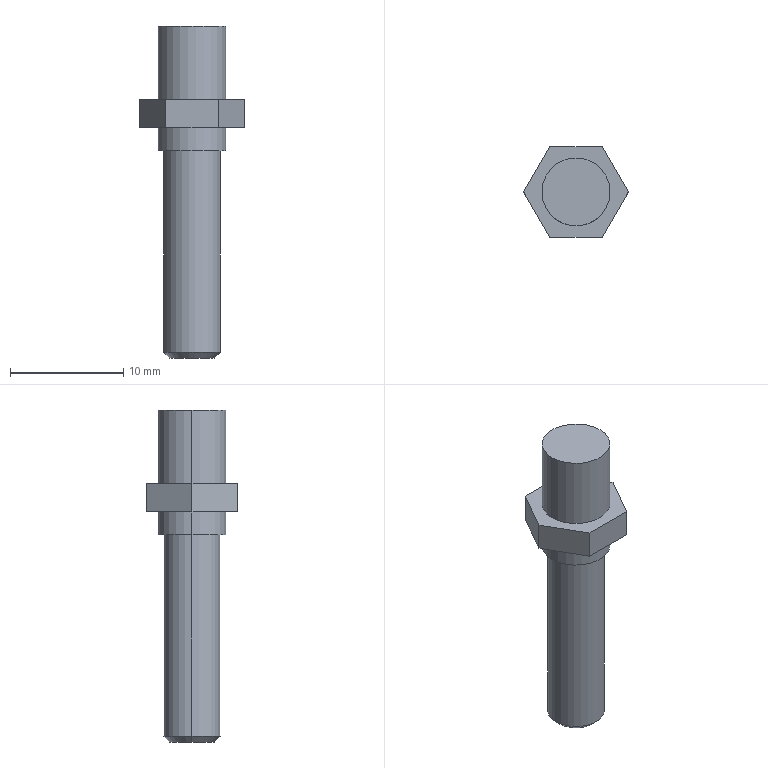Component | SolidWorks | CLS-MechanismAccessory5-1 | 1 solid | 19 faces | box 9.24 x 8 x 29.3 mm | volume 736 mm3 | plane 11 | cylinder 6 | cone 2 | commonest cylinder face diameters 6 x4 5 x2 | material 10 Cold Drawn Round Steel GB699-88
build123d program:
from build123d import *

# Parameters (mm, degrees)
BOSS_EXTRUDE1_DEPTH = 2.5
SKETCH2_R           = 3
BOSS_EXTRUDE2_DEPTH = 6.5
BOSS_EXTRUDE3_START = 2
SKETCH3_R           = 3
BOSS_EXTRUDE3_DEPTH = 2
SKETCH4_R           = 2.5
BOSS_EXTRUDE4_DEPTH = 18.3
CHAMFER1_SIZE       = 0.5


with BuildPart() as part:
    # Sketch1 → Boss-Extrude1 (new body)
    with BuildSketch(Plane.XY):
        Polygon((2.309, -4), (4.619, 0), (2.309, 4), (-2.309, 4), (-4.619, 0), (-2.309, -4), align=None)
    extrude(amount=BOSS_EXTRUDE1_DEPTH)

    # Sketch2 → Boss-Extrude2 (add)
    with BuildSketch(Plane.XY.offset(2.5)):
        with Locations(Location((0, 0, 0), (0, 0, 180))):
            Circle(SKETCH2_R)
    extrude(amount=BOSS_EXTRUDE2_DEPTH)

    # Sketch3 → Boss-Extrude3 (add)
    with BuildSketch(Plane(origin=(0, 0, 0), x_dir=(-1, 0, 0), z_dir=(0, 0, -1)).offset(BOSS_EXTRUDE3_START)):
        Circle(SKETCH3_R)
    extrude(amount=-BOSS_EXTRUDE3_DEPTH)

    # Sketch4 → Boss-Extrude4 (add)
    with BuildSketch(Plane(origin=(0, 0, -2), x_dir=(-1, 0, 0), z_dir=(0, 0, -1))):
        Circle(SKETCH4_R)
    extrude(amount=BOSS_EXTRUDE4_DEPTH)

    # Chamfer1
    chamfer1_edges = [part.edges().sort_by_distance(p)[0] for p in [
        (2.5, 0, -20.3),
    ]]
    chamfer(chamfer1_edges, length=CHAMFER1_SIZE)


solid = part.part

# Placed as in the assembly
solid = solid.moved(Location((63.64, 5.417, -1.001), (0, 0, 0)))
STEP:
#1=COLOUR_RGB('',0.7922,0.8196,0.9333);
#2=FILL_AREA_STYLE_COLOUR('',#1);
#3=FILL_AREA_STYLE('',(#2));
#4=SURFACE_STYLE_FILL_AREA(#3);
#5=SURFACE_SIDE_STYLE('',(#4));
#6=SURFACE_STYLE_USAGE(.BOTH.,#5);
#7=PRESENTATION_STYLE_ASSIGNMENT((#6));
#8=CARTESIAN_POINT('',(2.427,0.2133,-0.8386));
#9=VERTEX_POINT('',#8);
#10=CARTESIAN_POINT('',(2.584,0.2133,-0.8386));
#11=VERTEX_POINT('',#10);
#12=CARTESIAN_POINT('',(2.506,0.2133,-0.8386));
#13=DIRECTION('',(0.,0.,-1.));
#14=DIRECTION('',(-1.,0.,0.));
#15=AXIS2_PLACEMENT_3D('',#12,#13,#14);
#16=CIRCLE('',#15,0.07874);
#17=EDGE_CURVE('',#9,#11,#16,.T.);
#18=ORIENTED_EDGE('',*,*,#17,.F.);
#19=CARTESIAN_POINT('',(2.407,0.2133,-0.8189));
#20=VERTEX_POINT('',#19);
#21=CARTESIAN_POINT('',(2.427,0.2133,-0.8386));
#22=DIRECTION('',(-0.7071,0.,0.7071));
#23=VECTOR('',#22,39.37);
#24=LINE('',#21,#23);
#25=EDGE_CURVE('',#9,#20,#24,.T.);
#26=ORIENTED_EDGE('',*,*,#25,.T.);
#27=CARTESIAN_POINT('',(2.604,0.2133,-0.8189));
#28=VERTEX_POINT('',#27);
#29=CARTESIAN_POINT('',(2.506,0.2133,-0.8189));
#30=DIRECTION('',(0.,0.,1.));
#31=DIRECTION('',(-1.,0.,0.));
#32=AXIS2_PLACEMENT_3D('',#29,#30,#31);
#33=CIRCLE('',#32,0.09843);
#34=EDGE_CURVE('',#28,#20,#33,.T.);
#35=ORIENTED_EDGE('',*,*,#34,.F.);
#36=CARTESIAN_POINT('',(2.584,0.2133,-0.8386));
#37=DIRECTION('',(0.7071,0.,0.7071));
#38=VECTOR('',#37,39.37);
#39=LINE('',#36,#38);
#40=EDGE_CURVE('',#11,#28,#39,.T.);
#41=ORIENTED_EDGE('',*,*,#40,.F.);
#42=EDGE_LOOP('',(#18,#26,#35,#41));
#43=FACE_OUTER_BOUND('',#42,.T.);
#44=CARTESIAN_POINT('',(2.506,0.2133,-0.8386));
#45=DIRECTION('',(0.,0.,1.));
#46=DIRECTION('',(1.,0.,0.));
#47=AXIS2_PLACEMENT_3D('',#44,#45,#46);
#48=CONICAL_SURFACE('',#47,0.07874,0.7854);
#49=ADVANCED_FACE('',(#43),#48,.T.);
#50=ORIENTED_EDGE('',*,*,#34,.T.);
#51=CARTESIAN_POINT('',(2.407,0.2133,-0.1181));
#52=VERTEX_POINT('',#51);
#53=CARTESIAN_POINT('',(2.407,0.2133,-0.8386));
#54=DIRECTION('',(0.,0.,1.));
#55=VECTOR('',#54,39.37);
#56=LINE('',#53,#55);
#57=EDGE_CURVE('',#20,#52,#56,.T.);
#58=ORIENTED_EDGE('',*,*,#57,.T.);
#59=CARTESIAN_POINT('',(2.604,0.2133,-0.1181));
#60=VERTEX_POINT('',#59);
#61=CARTESIAN_POINT('',(2.506,0.2133,-0.1181));
#62=DIRECTION('',(0.,0.,-1.));
#63=DIRECTION('',(-1.,0.,0.));
#64=AXIS2_PLACEMENT_3D('',#61,#62,#63);
#65=CIRCLE('',#64,0.09843);
#66=EDGE_CURVE('',#52,#60,#65,.T.);
#67=ORIENTED_EDGE('',*,*,#66,.T.);
#68=CARTESIAN_POINT('',(2.604,0.2133,-0.8386));
#69=DIRECTION('',(0.,0.,1.));
#70=VECTOR('',#69,39.37);
#71=LINE('',#68,#70);
#72=EDGE_CURVE('',#28,#60,#71,.T.);
#73=ORIENTED_EDGE('',*,*,#72,.F.);
#74=EDGE_LOOP('',(#50,#58,#67,#73));
#75=FACE_OUTER_BOUND('',#74,.T.);
#76=CARTESIAN_POINT('',(2.506,0.2133,-0.8386));
#77=DIRECTION('',(0.,0.,1.));
#78=DIRECTION('',(1.,0.,0.));
#79=AXIS2_PLACEMENT_3D('',#76,#77,#78);
#80=CYLINDRICAL_SURFACE('',#79,0.09843);
#81=ADVANCED_FACE('',(#75),#80,.T.);
#82=CARTESIAN_POINT('',(2.387,0.2133,-0.1181));
#83=VERTEX_POINT('',#82);
#84=CARTESIAN_POINT('',(2.624,0.2133,-0.1181));
#85=VERTEX_POINT('',#84);
#86=CARTESIAN_POINT('',(2.506,0.2133,-0.1181));
#87=DIRECTION('',(0.,0.,-1.));
#88=DIRECTION('',(-1.,0.,0.));
#89=AXIS2_PLACEMENT_3D('',#86,#87,#88);
#90=CIRCLE('',#89,0.1181);
#91=EDGE_CURVE('',#83,#85,#90,.T.);
#92=ORIENTED_EDGE('',*,*,#91,.F.);
#93=CARTESIAN_POINT('',(2.387,0.2133,-0.03939));
#94=VERTEX_POINT('',#93);
#95=CARTESIAN_POINT('',(2.387,0.2133,-0.1181));
#96=DIRECTION('',(0.,0.,1.));
#97=VECTOR('',#96,39.37);
#98=LINE('',#95,#97);
#99=EDGE_CURVE('',#83,#94,#98,.T.);
#100=ORIENTED_EDGE('',*,*,#99,.T.);
#101=CARTESIAN_POINT('',(2.624,0.2133,-0.03939));
#102=VERTEX_POINT('',#101);
#103=CARTESIAN_POINT('',(2.506,0.2133,-0.03939));
#104=DIRECTION('',(0.,0.,-1.));
#105=DIRECTION('',(1.,0.,0.));
#106=AXIS2_PLACEMENT_3D('',#103,#104,#105);
#107=CIRCLE('',#106,0.1181);
#108=EDGE_CURVE('',#94,#102,#107,.T.);
#109=ORIENTED_EDGE('',*,*,#108,.T.);
#110=CARTESIAN_POINT('',(2.624,0.2133,-0.1181));
#111=DIRECTION('',(0.,0.,1.));
#112=VECTOR('',#111,39.37);
#113=LINE('',#110,#112);
#114=EDGE_CURVE('',#85,#102,#113,.T.);
#115=ORIENTED_EDGE('',*,*,#114,.F.);
#116=EDGE_LOOP('',(#92,#100,#109,#115));
#117=FACE_OUTER_BOUND('',#116,.T.);
#118=CARTESIAN_POINT('',(2.506,0.2133,-0.1181));
#119=DIRECTION('',(0.,0.,1.));
#120=DIRECTION('',(1.,0.,0.));
#121=AXIS2_PLACEMENT_3D('',#118,#119,#120);
#122=CYLINDRICAL_SURFACE('',#121,0.1181);
#123=ADVANCED_FACE('',(#117),#122,.T.);
#124=CARTESIAN_POINT('',(2.624,0.2133,0.3149));
#125=VERTEX_POINT('',#124);
#126=CARTESIAN_POINT('',(2.387,0.2133,0.3149));
#127=VERTEX_POINT('',#126);
#128=CARTESIAN_POINT('',(2.506,0.2133,0.3149));
#129=DIRECTION('',(0.,0.,1.));
#130=DIRECTION('',(1.,0.,0.));
#131=AXIS2_PLACEMENT_3D('',#128,#129,#130);
#132=CIRCLE('',#131,0.1181);
#133=EDGE_CURVE('',#125,#127,#132,.T.);
#134=ORIENTED_EDGE('',*,*,#133,.F.);
#135=CARTESIAN_POINT('',(2.624,0.2133,0.05903));
#136=VERTEX_POINT('',#135);
#137=CARTESIAN_POINT('',(2.624,0.2133,0.3149));
#138=DIRECTION('',(0.,0.,-1.));
#139=VECTOR('',#138,39.37);
#140=LINE('',#137,#139);
#141=EDGE_CURVE('',#125,#136,#140,.T.);
#142=ORIENTED_EDGE('',*,*,#141,.T.);
#143=CARTESIAN_POINT('',(2.387,0.2133,0.05903));
#144=VERTEX_POINT('',#143);
#145=CARTESIAN_POINT('',(2.506,0.2133,0.05903));
#146=DIRECTION('',(0.,0.,1.));
#147=DIRECTION('',(1.,0.,0.));
#148=AXIS2_PLACEMENT_3D('',#145,#146,#147);
#149=CIRCLE('',#148,0.1181);
#150=EDGE_CURVE('',#136,#144,#149,.T.);
#151=ORIENTED_EDGE('',*,*,#150,.T.);
#152=CARTESIAN_POINT('',(2.387,0.2133,0.3149));
#153=DIRECTION('',(0.,0.,-1.));
#154=VECTOR('',#153,39.37);
#155=LINE('',#152,#154);
#156=EDGE_CURVE('',#127,#144,#155,.T.);
#157=ORIENTED_EDGE('',*,*,#156,.F.);
#158=EDGE_LOOP('',(#134,#142,#151,#157));
#159=FACE_OUTER_BOUND('',#158,.T.);
#160=CARTESIAN_POINT('',(2.506,0.2133,0.3149));
#161=DIRECTION('',(0.,0.,-1.));
#162=DIRECTION('',(-1.,0.,0.));
#163=AXIS2_PLACEMENT_3D('',#160,#161,#162);
#164=CYLINDRICAL_SURFACE('',#163,0.1181);
#165=ADVANCED_FACE('',(#159),#164,.T.);
#166=CARTESIAN_POINT('',(2.506,0.2133,-0.1181));
#167=DIRECTION('',(0.,0.,-1.));
#168=DIRECTION('',(-1.,0.,0.));
#169=AXIS2_PLACEMENT_3D('',#166,#167,#168);
#170=CIRCLE('',#169,0.1181);
#171=EDGE_CURVE('',#85,#83,#170,.T.);
#172=ORIENTED_EDGE('',*,*,#171,.T.);
#173=ORIENTED_EDGE('',*,*,#91,.T.);
#174=EDGE_LOOP('',(#172,#173));
#175=FACE_OUTER_BOUND('',#174,.T.);
#176=CARTESIAN_POINT('',(2.506,0.2133,-0.1181));
#177=DIRECTION('',(0.,0.,-1.));
#178=DIRECTION('',(-1.,0.,0.));
#179=AXIS2_PLACEMENT_3D('',#176,#177,#178);
#180=CIRCLE('',#179,0.09843);
#181=EDGE_CURVE('',#60,#52,#180,.T.);
#182=ORIENTED_EDGE('',*,*,#181,.F.);
#183=ORIENTED_EDGE('',*,*,#66,.F.);
#184=EDGE_LOOP('',(#182,#183));
#185=FACE_BOUND('',#184,.T.);
#186=CARTESIAN_POINT('',(2.506,0.2133,-0.1181));
#187=DIRECTION('',(0.,0.,-1.));
#188=DIRECTION('',(-1.,0.,0.));
#189=AXIS2_PLACEMENT_3D('',#186,#187,#188);
#190=PLANE('',#189);
#191=ADVANCED_FACE('',(#175,#185),#190,.T.);
#192=CARTESIAN_POINT('',(2.415,0.05578,-0.03939));
#193=VERTEX_POINT('',#192);
#194=CARTESIAN_POINT('',(2.596,0.05578,-0.03939));
#195=VERTEX_POINT('',#194);
#196=CARTESIAN_POINT('',(2.415,0.05578,-0.03939));
#197=DIRECTION('',(1.,0.,0.));
#198=VECTOR('',#197,39.37);
#199=LINE('',#196,#198);
#200=EDGE_CURVE('',#193,#195,#199,.T.);
#201=ORIENTED_EDGE('',*,*,#200,.F.);
#202=CARTESIAN_POINT('',(2.324,0.2133,-0.03939));
#203=VERTEX_POINT('',#202);
#204=CARTESIAN_POINT('',(2.324,0.2133,-0.03939));
#205=DIRECTION('',(0.5,-0.866,0.));
#206=VECTOR('',#205,39.37);
#207=LINE('',#204,#206);
#208=EDGE_CURVE('',#203,#193,#207,.T.);
#209=ORIENTED_EDGE('',*,*,#208,.F.);
#210=CARTESIAN_POINT('',(2.415,0.3707,-0.03939));
#211=VERTEX_POINT('',#210);
#212=CARTESIAN_POINT('',(2.415,0.3707,-0.03939));
#213=DIRECTION('',(-0.5,-0.866,0.));
#214=VECTOR('',#213,39.37);
#215=LINE('',#212,#214);
#216=EDGE_CURVE('',#211,#203,#215,.T.);
#217=ORIENTED_EDGE('',*,*,#216,.F.);
#218=CARTESIAN_POINT('',(2.596,0.3707,-0.03939));
#219=VERTEX_POINT('',#218);
#220=CARTESIAN_POINT('',(2.596,0.3707,-0.03939));
#221=DIRECTION('',(-1.,-0.,0.));
#222=VECTOR('',#221,39.37);
#223=LINE('',#220,#222);
#224=EDGE_CURVE('',#219,#211,#223,.T.);
#225=ORIENTED_EDGE('',*,*,#224,.F.);
#226=CARTESIAN_POINT('',(2.687,0.2133,-0.03939));
#227=VERTEX_POINT('',#226);
#228=CARTESIAN_POINT('',(2.687,0.2133,-0.03939));
#229=DIRECTION('',(-0.5,0.866,0.));
#230=VECTOR('',#229,39.37);
#231=LINE('',#228,#230);
#232=EDGE_CURVE('',#227,#219,#231,.T.);
#233=ORIENTED_EDGE('',*,*,#232,.F.);
#234=CARTESIAN_POINT('',(2.596,0.05578,-0.03939));
#235=DIRECTION('',(0.5,0.866,0.));
#236=VECTOR('',#235,39.37);
#237=LINE('',#234,#236);
#238=EDGE_CURVE('',#195,#227,#237,.T.);
#239=ORIENTED_EDGE('',*,*,#238,.F.);
#240=EDGE_LOOP('',(#201,#209,#217,#225,#233,#239));
#241=FACE_OUTER_BOUND('',#240,.T.);
#242=CARTESIAN_POINT('',(2.506,0.2133,-0.03939));
#243=DIRECTION('',(0.,0.,-1.));
#244=DIRECTION('',(1.,0.,0.));
#245=AXIS2_PLACEMENT_3D('',#242,#243,#244);
#246=CIRCLE('',#245,0.1181);
#247=EDGE_CURVE('',#102,#94,#246,.T.);
#248=ORIENTED_EDGE('',*,*,#247,.F.);
#249=ORIENTED_EDGE('',*,*,#108,.F.);
#250=EDGE_LOOP('',(#248,#249));
#251=FACE_BOUND('',#250,.T.);
#252=CARTESIAN_POINT('',(2.596,0.05578,-0.03939));
#253=DIRECTION('',(0.,0.,1.));
#254=DIRECTION('',(1.,0.,0.));
#255=AXIS2_PLACEMENT_3D('',#252,#253,#254);
#256=PLANE('',#255);
#257=ADVANCED_FACE('',(#241,#251),#256,.F.);
#258=CARTESIAN_POINT('',(2.415,0.05578,0.05903));
#259=VERTEX_POINT('',#258);
#260=CARTESIAN_POINT('',(2.596,0.05578,0.05903));
#261=VERTEX_POINT('',#260);
#262=CARTESIAN_POINT('',(2.415,0.05578,0.05903));
#263=DIRECTION('',(1.,0.,0.));
#264=VECTOR('',#263,39.37);
#265=LINE('',#262,#264);
#266=EDGE_CURVE('',#259,#261,#265,.T.);
#267=ORIENTED_EDGE('',*,*,#266,.T.);
#268=CARTESIAN_POINT('',(2.687,0.2133,0.05903));
#269=VERTEX_POINT('',#268);
#270=CARTESIAN_POINT('',(2.596,0.05578,0.05903));
#271=DIRECTION('',(0.5,0.866,0.));
#272=VECTOR('',#271,39.37);
#273=LINE('',#270,#272);
#274=EDGE_CURVE('',#261,#269,#273,.T.);
#275=ORIENTED_EDGE('',*,*,#274,.T.);
#276=CARTESIAN_POINT('',(2.596,0.3707,0.05903));
#277=VERTEX_POINT('',#276);
#278=CARTESIAN_POINT('',(2.687,0.2133,0.05903));
#279=DIRECTION('',(-0.5,0.866,0.));
#280=VECTOR('',#279,39.37);
#281=LINE('',#278,#280);
#282=EDGE_CURVE('',#269,#277,#281,.T.);
#283=ORIENTED_EDGE('',*,*,#282,.T.);
#284=CARTESIAN_POINT('',(2.415,0.3707,0.05903));
#285=VERTEX_POINT('',#284);
#286=CARTESIAN_POINT('',(2.596,0.3707,0.05903));
#287=DIRECTION('',(-1.,-0.,0.));
#288=VECTOR('',#287,39.37);
#289=LINE('',#286,#288);
#290=EDGE_CURVE('',#277,#285,#289,.T.);
#291=ORIENTED_EDGE('',*,*,#290,.T.);
#292=CARTESIAN_POINT('',(2.324,0.2133,0.05903));
#293=VERTEX_POINT('',#292);
#294=CARTESIAN_POINT('',(2.415,0.3707,0.05903));
#295=DIRECTION('',(-0.5,-0.866,0.));
#296=VECTOR('',#295,39.37);
#297=LINE('',#294,#296);
#298=EDGE_CURVE('',#285,#293,#297,.T.);
#299=ORIENTED_EDGE('',*,*,#298,.T.);
#300=CARTESIAN_POINT('',(2.324,0.2133,0.05903));
#301=DIRECTION('',(0.5,-0.866,0.));
#302=VECTOR('',#301,39.37);
#303=LINE('',#300,#302);
#304=EDGE_CURVE('',#293,#259,#303,.T.);
#305=ORIENTED_EDGE('',*,*,#304,.T.);
#306=EDGE_LOOP('',(#267,#275,#283,#291,#299,#305));
#307=FACE_OUTER_BOUND('',#306,.T.);
#308=CARTESIAN_POINT('',(2.506,0.2133,0.05903));
#309=DIRECTION('',(0.,0.,1.));
#310=DIRECTION('',(1.,0.,0.));
#311=AXIS2_PLACEMENT_3D('',#308,#309,#310);
#312=CIRCLE('',#311,0.1181);
#313=EDGE_CURVE('',#144,#136,#312,.T.);
#314=ORIENTED_EDGE('',*,*,#313,.F.);
#315=ORIENTED_EDGE('',*,*,#150,.F.);
#316=EDGE_LOOP('',(#314,#315));
#317=FACE_BOUND('',#316,.T.);
#318=CARTESIAN_POINT('',(2.596,0.05578,0.05903));
#319=DIRECTION('',(0.,0.,1.));
#320=DIRECTION('',(1.,0.,0.));
#321=AXIS2_PLACEMENT_3D('',#318,#319,#320);
#322=PLANE('',#321);
#323=ADVANCED_FACE('',(#307,#317),#322,.T.);
#324=ORIENTED_EDGE('',*,*,#200,.T.);
#325=CARTESIAN_POINT('',(2.596,0.05578,0.05903));
#326=DIRECTION('',(0.,0.,-1.));
#327=VECTOR('',#326,39.37);
#328=LINE('',#325,#327);
#329=EDGE_CURVE('',#261,#195,#328,.T.);
#330=ORIENTED_EDGE('',*,*,#329,.F.);
#331=ORIENTED_EDGE('',*,*,#266,.F.);
#332=CARTESIAN_POINT('',(2.415,0.05578,0.05903));
#333=DIRECTION('',(0.,0.,-1.));
#334=VECTOR('',#333,39.37);
#335=LINE('',#332,#334);
#336=EDGE_CURVE('',#259,#193,#335,.T.);
#337=ORIENTED_EDGE('',*,*,#336,.T.);
#338=EDGE_LOOP('',(#324,#330,#331,#337));
#339=FACE_OUTER_BOUND('',#338,.T.);
#340=CARTESIAN_POINT('',(2.415,0.05578,0.05903));
#341=DIRECTION('',(0.,1.,0.));
#342=DIRECTION('',(0.,0.,1.));
#343=AXIS2_PLACEMENT_3D('',#340,#341,#342);
#344=PLANE('',#343);
#345=ADVANCED_FACE('',(#339),#344,.F.);
#346=ORIENTED_EDGE('',*,*,#238,.T.);
#347=CARTESIAN_POINT('',(2.687,0.2133,0.05903));
#348=DIRECTION('',(0.,0.,-1.));
#349=VECTOR('',#348,39.37);
#350=LINE('',#347,#349);
#351=EDGE_CURVE('',#269,#227,#350,.T.);
#352=ORIENTED_EDGE('',*,*,#351,.F.);
#353=ORIENTED_EDGE('',*,*,#274,.F.);
#354=ORIENTED_EDGE('',*,*,#329,.T.);
#355=EDGE_LOOP('',(#346,#352,#353,#354));
#356=FACE_OUTER_BOUND('',#355,.T.);
#357=CARTESIAN_POINT('',(2.596,0.05578,0.05903));
#358=DIRECTION('',(-0.866,0.5,0.));
#359=DIRECTION('',(-0.5,-0.866,0.));
#360=AXIS2_PLACEMENT_3D('',#357,#358,#359);
#361=PLANE('',#360);
#362=ADVANCED_FACE('',(#356),#361,.F.);
#363=ORIENTED_EDGE('',*,*,#232,.T.);
#364=CARTESIAN_POINT('',(2.596,0.3707,0.05903));
#365=DIRECTION('',(0.,0.,-1.));
#366=VECTOR('',#365,39.37);
#367=LINE('',#364,#366);
#368=EDGE_CURVE('',#277,#219,#367,.T.);
#369=ORIENTED_EDGE('',*,*,#368,.F.);
#370=ORIENTED_EDGE('',*,*,#282,.F.);
#371=ORIENTED_EDGE('',*,*,#351,.T.);
#372=EDGE_LOOP('',(#363,#369,#370,#371));
#373=FACE_OUTER_BOUND('',#372,.T.);
#374=CARTESIAN_POINT('',(2.687,0.2133,0.05903));
#375=DIRECTION('',(-0.866,-0.5,0.));
#376=DIRECTION('',(0.5,-0.866,0.));
#377=AXIS2_PLACEMENT_3D('',#374,#375,#376);
#378=PLANE('',#377);
#379=ADVANCED_FACE('',(#373),#378,.F.);
#380=ORIENTED_EDGE('',*,*,#224,.T.);
#381=CARTESIAN_POINT('',(2.415,0.3707,0.05903));
#382=DIRECTION('',(0.,0.,-1.));
#383=VECTOR('',#382,39.37);
#384=LINE('',#381,#383);
#385=EDGE_CURVE('',#285,#211,#384,.T.);
#386=ORIENTED_EDGE('',*,*,#385,.F.);
#387=ORIENTED_EDGE('',*,*,#290,.F.);
#388=ORIENTED_EDGE('',*,*,#368,.T.);
#389=EDGE_LOOP('',(#380,#386,#387,#388));
#390=FACE_OUTER_BOUND('',#389,.T.);
#391=CARTESIAN_POINT('',(2.596,0.3707,0.05903));
#392=DIRECTION('',(0.,-1.,0.));
#393=DIRECTION('',(1.,0.,0.));
#394=AXIS2_PLACEMENT_3D('',#391,#392,#393);
#395=PLANE('',#394);
#396=ADVANCED_FACE('',(#390),#395,.F.);
#397=ORIENTED_EDGE('',*,*,#216,.T.);
#398=CARTESIAN_POINT('',(2.324,0.2133,0.05903));
#399=DIRECTION('',(0.,0.,-1.));
#400=VECTOR('',#399,39.37);
#401=LINE('',#398,#400);
#402=EDGE_CURVE('',#293,#203,#401,.T.);
#403=ORIENTED_EDGE('',*,*,#402,.F.);
#404=ORIENTED_EDGE('',*,*,#298,.F.);
#405=ORIENTED_EDGE('',*,*,#385,.T.);
#406=EDGE_LOOP('',(#397,#403,#404,#405));
#407=FACE_OUTER_BOUND('',#406,.T.);
#408=CARTESIAN_POINT('',(2.415,0.3707,0.05903));
#409=DIRECTION('',(0.866,-0.5,0.));
#410=DIRECTION('',(0.5,0.866,0.));
#411=AXIS2_PLACEMENT_3D('',#408,#409,#410);
#412=PLANE('',#411);
#413=ADVANCED_FACE('',(#407),#412,.F.);
#414=ORIENTED_EDGE('',*,*,#208,.T.);
#415=ORIENTED_EDGE('',*,*,#336,.F.);
#416=ORIENTED_EDGE('',*,*,#304,.F.);
#417=ORIENTED_EDGE('',*,*,#402,.T.);
#418=EDGE_LOOP('',(#414,#415,#416,#417));
#419=FACE_OUTER_BOUND('',#418,.T.);
#420=CARTESIAN_POINT('',(2.324,0.2133,0.05903));
#421=DIRECTION('',(0.866,0.5,0.));
#422=DIRECTION('',(-0.5,0.866,0.));
#423=AXIS2_PLACEMENT_3D('',#420,#421,#422);
#424=PLANE('',#423);
#425=ADVANCED_FACE('',(#419),#424,.F.);
#426=ORIENTED_EDGE('',*,*,#141,.F.);
#427=CARTESIAN_POINT('',(2.506,0.2133,0.3149));
#428=DIRECTION('',(0.,0.,1.));
#429=DIRECTION('',(1.,0.,0.));
#430=AXIS2_PLACEMENT_3D('',#427,#428,#429);
#431=CIRCLE('',#430,0.1181);
#432=EDGE_CURVE('',#127,#125,#431,.T.);
#433=ORIENTED_EDGE('',*,*,#432,.F.);
#434=ORIENTED_EDGE('',*,*,#156,.T.);
#435=ORIENTED_EDGE('',*,*,#313,.T.);
#436=EDGE_LOOP('',(#426,#433,#434,#435));
#437=FACE_OUTER_BOUND('',#436,.T.);
#438=CARTESIAN_POINT('',(2.506,0.2133,0.3149));
#439=DIRECTION('',(0.,0.,-1.));
#440=DIRECTION('',(-1.,0.,0.));
#441=AXIS2_PLACEMENT_3D('',#438,#439,#440);
#442=CYLINDRICAL_SURFACE('',#441,0.1181);
#443=ADVANCED_FACE('',(#437),#442,.T.);
#444=ORIENTED_EDGE('',*,*,#432,.T.);
#445=ORIENTED_EDGE('',*,*,#133,.T.);
#446=EDGE_LOOP('',(#444,#445));
#447=FACE_OUTER_BOUND('',#446,.T.);
#448=CARTESIAN_POINT('',(2.506,0.2133,0.3149));
#449=DIRECTION('',(0.,0.,1.));
#450=DIRECTION('',(1.,0.,0.));
#451=AXIS2_PLACEMENT_3D('',#448,#449,#450);
#452=PLANE('',#451);
#453=ADVANCED_FACE('',(#447),#452,.T.);
#454=ORIENTED_EDGE('',*,*,#99,.F.);
#455=ORIENTED_EDGE('',*,*,#171,.F.);
#456=ORIENTED_EDGE('',*,*,#114,.T.);
#457=ORIENTED_EDGE('',*,*,#247,.T.);
#458=EDGE_LOOP('',(#454,#455,#456,#457));
#459=FACE_OUTER_BOUND('',#458,.T.);
#460=CARTESIAN_POINT('',(2.506,0.2133,-0.1181));
#461=DIRECTION('',(0.,0.,1.));
#462=DIRECTION('',(1.,0.,0.));
#463=AXIS2_PLACEMENT_3D('',#460,#461,#462);
#464=CYLINDRICAL_SURFACE('',#463,0.1181);
#465=ADVANCED_FACE('',(#459),#464,.T.);
#466=ORIENTED_EDGE('',*,*,#57,.F.);
#467=CARTESIAN_POINT('',(2.506,0.2133,-0.8189));
#468=DIRECTION('',(0.,0.,1.));
#469=DIRECTION('',(-1.,0.,0.));
#470=AXIS2_PLACEMENT_3D('',#467,#468,#469);
#471=CIRCLE('',#470,0.09843);
#472=EDGE_CURVE('',#20,#28,#471,.T.);
#473=ORIENTED_EDGE('',*,*,#472,.T.);
#474=ORIENTED_EDGE('',*,*,#72,.T.);
#475=ORIENTED_EDGE('',*,*,#181,.T.);
#476=EDGE_LOOP('',(#466,#473,#474,#475));
#477=FACE_OUTER_BOUND('',#476,.T.);
#478=CARTESIAN_POINT('',(2.506,0.2133,-0.8386));
#479=DIRECTION('',(0.,0.,1.));
#480=DIRECTION('',(1.,0.,0.));
#481=AXIS2_PLACEMENT_3D('',#478,#479,#480);
#482=CYLINDRICAL_SURFACE('',#481,0.09843);
#483=ADVANCED_FACE('',(#477),#482,.T.);
#484=CARTESIAN_POINT('',(2.506,0.2133,-0.8386));
#485=DIRECTION('',(0.,0.,-1.));
#486=DIRECTION('',(-1.,0.,0.));
#487=AXIS2_PLACEMENT_3D('',#484,#485,#486);
#488=CIRCLE('',#487,0.07874);
#489=EDGE_CURVE('',#11,#9,#488,.T.);
#490=ORIENTED_EDGE('',*,*,#489,.T.);
#491=ORIENTED_EDGE('',*,*,#17,.T.);
#492=EDGE_LOOP('',(#490,#491));
#493=FACE_OUTER_BOUND('',#492,.T.);
#494=CARTESIAN_POINT('',(2.506,0.2133,-0.8386));
#495=DIRECTION('',(0.,0.,-1.));
#496=DIRECTION('',(-1.,0.,0.));
#497=AXIS2_PLACEMENT_3D('',#494,#495,#496);
#498=PLANE('',#497);
#499=ADVANCED_FACE('',(#493),#498,.T.);
#500=ORIENTED_EDGE('',*,*,#25,.F.);
#501=ORIENTED_EDGE('',*,*,#489,.F.);
#502=ORIENTED_EDGE('',*,*,#40,.T.);
#503=ORIENTED_EDGE('',*,*,#472,.F.);
#504=EDGE_LOOP('',(#500,#501,#502,#503));
#505=FACE_OUTER_BOUND('',#504,.T.);
#506=CARTESIAN_POINT('',(2.506,0.2133,-0.8386));
#507=DIRECTION('',(0.,0.,1.));
#508=DIRECTION('',(1.,0.,0.));
#509=AXIS2_PLACEMENT_3D('',#506,#507,#508);
#510=CONICAL_SURFACE('',#509,0.07874,0.7854);
#511=ADVANCED_FACE('',(#505),#510,.T.);
#512=CLOSED_SHELL('',(#49,#81,#123,#165,#191,#257,#323,#345,#362,#379,#396,#413,#425,#443,#453,#465,#483,#499,#511));
#513=MANIFOLD_SOLID_BREP('',#512);
#514=STYLED_ITEM('',(#7),#513);
#515=(LENGTH_UNIT()NAMED_UNIT(*)SI_UNIT($,.METRE.));
#516=LENGTH_MEASURE_WITH_UNIT(LENGTH_MEASURE(0.0254),#515);
#517=DIMENSIONAL_EXPONENTS(1.,0.,0.,0.,0.,0.,0.);
#518=(CONVERSION_BASED_UNIT('',#516)LENGTH_UNIT()NAMED_UNIT(#517));
#519=UNCERTAINTY_MEASURE_WITH_UNIT(LENGTH_MEASURE(0.00001),#518,'','');
#520=(NAMED_UNIT(*)PLANE_ANGLE_UNIT()SI_UNIT($,.RADIAN.));
#521=(NAMED_UNIT(*)SI_UNIT($,.STERADIAN.)SOLID_ANGLE_UNIT());
#522=(GEOMETRIC_REPRESENTATION_CONTEXT(3)GLOBAL_UNCERTAINTY_ASSIGNED_CONTEXT((#519))GLOBAL_UNIT_ASSIGNED_CONTEXT((#518,#520,#521))REPRESENTATION_CONTEXT('',''));
#523=MECHANICAL_DESIGN_GEOMETRIC_PRESENTATION_REPRESENTATION('',(#514),#522);
#524=CARTESIAN_POINT('',(0.,0.,0.));
#525=DIRECTION('',(0.,0.,1.));
#526=DIRECTION('',(1.,0.,0.));
#527=AXIS2_PLACEMENT_3D('',#524,#525,#526);
#528=(LENGTH_UNIT()NAMED_UNIT(*)SI_UNIT($,.METRE.));
#529=LENGTH_MEASURE_WITH_UNIT(LENGTH_MEASURE(0.0254),#528);
#530=DIMENSIONAL_EXPONENTS(1.,0.,0.,0.,0.,0.,0.);
#531=(CONVERSION_BASED_UNIT('',#529)LENGTH_UNIT()NAMED_UNIT(#530));
#532=UNCERTAINTY_MEASURE_WITH_UNIT(LENGTH_MEASURE(0.00001),#531,'','');
#533=(NAMED_UNIT(*)PLANE_ANGLE_UNIT()SI_UNIT($,.RADIAN.));
#534=(NAMED_UNIT(*)SI_UNIT($,.STERADIAN.)SOLID_ANGLE_UNIT());
#535=(GEOMETRIC_REPRESENTATION_CONTEXT(3)GLOBAL_UNCERTAINTY_ASSIGNED_CONTEXT((#532))GLOBAL_UNIT_ASSIGNED_CONTEXT((#531,#533,#534))REPRESENTATION_CONTEXT('',''));
#536=ADVANCED_BREP_SHAPE_REPRESENTATION('',(#513,#527),#535);
#537=PRESENTATION_LAYER_ASSIGNMENT('','',(#514));